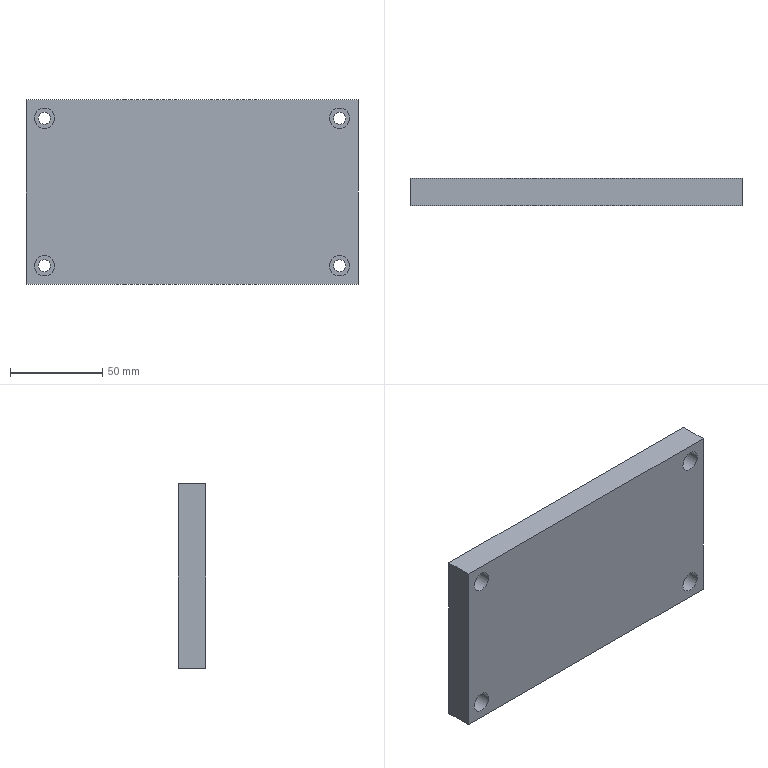Component | SolidWorks | SHYTJ-01-03-05-1 | 1 solid | 26 faces | box 180 x 15 x 100 mm | volume 266001 mm3 | cylinder 16 | plane 10 | commonest cylinder face diameters 11 x8 6.6 x8
build123d program:
from build123d import *

# Parameters (mm, degrees)
SKETCH1_W                                         = 180
SKETCH1_H                                         = 100
BOSS_EXTRUDE1_DEPTH                               = 15
HOLE_SIZE_ACCORDING_TO_TYPE_OF_SOCKET_D           = 6.6
HOLE_SIZE_ACCORDING_TO_TYPE_OF_SOCKET_DEPTH       = 19.75
HOLE_SIZE_ACCORDING_TO_TYPE_OF_SOCKET_CBORE_D     = 11
HOLE_SIZE_ACCORDING_TO_TYPE_OF_SOCKET_CBORE_DEPTH = 8
HOLE_SIZE_ACCORDING_TO_TYPE_OF_SOCKET_TIP         = 1.983


with BuildPart() as part:
    # Sketch1 → Boss-Extrude1 (new body)
    with BuildSketch(Plane.XY):
        with Locations((-90, -50)):
            Rectangle(SKETCH1_W, SKETCH1_H)
    extrude(amount=BOSS_EXTRUDE1_DEPTH)

    # Hole Size _according to_ type of socket
    with Locations(Plane(origin=(0, 0, 0), x_dir=(-1, 0, 0), z_dir=(0, 0, -1))):
        with Locations((10, -10), (10, -90), (170, -90), (170, -10)):
            CounterBoreHole(HOLE_SIZE_ACCORDING_TO_TYPE_OF_SOCKET_D / 2, HOLE_SIZE_ACCORDING_TO_TYPE_OF_SOCKET_CBORE_D / 2, HOLE_SIZE_ACCORDING_TO_TYPE_OF_SOCKET_CBORE_DEPTH, depth=HOLE_SIZE_ACCORDING_TO_TYPE_OF_SOCKET_DEPTH)
            with Locations((0, 0, -(HOLE_SIZE_ACCORDING_TO_TYPE_OF_SOCKET_DEPTH + HOLE_SIZE_ACCORDING_TO_TYPE_OF_SOCKET_TIP / 2))):  # 118° drill point
                Cone(0, HOLE_SIZE_ACCORDING_TO_TYPE_OF_SOCKET_D / 2, HOLE_SIZE_ACCORDING_TO_TYPE_OF_SOCKET_TIP, mode=Mode.SUBTRACT)


solid = part.part

# Placed as in the assembly
solid = solid.moved(Location((115.884, -80.361, 220), (-90, 0, 0)))
STEP:
#1=CARTESIAN_POINT('',(4.385,-2.849,9.055));
#2=VERTEX_POINT('',#1);
#3=CARTESIAN_POINT('',(3.952,-2.849,9.055));
#4=VERTEX_POINT('',#3);
#5=CARTESIAN_POINT('',(4.169,-2.849,9.055));
#6=DIRECTION('',(-0.,-1.,-0.));
#7=DIRECTION('',(-1.,0.,0.));
#8=AXIS2_PLACEMENT_3D('',#5,#6,#7);
#9=CIRCLE('',#8,0.2165);
#10=EDGE_CURVE('',#2,#4,#9,.T.);
#11=ORIENTED_EDGE('',*,*,#10,.F.);
#12=CARTESIAN_POINT('',(4.385,-3.164,9.055));
#13=VERTEX_POINT('',#12);
#14=CARTESIAN_POINT('',(4.385,-3.164,9.055));
#15=DIRECTION('',(-0.,-1.,-0.));
#16=VECTOR('',#15,39.37);
#17=LINE('',#14,#16);
#18=EDGE_CURVE('',#2,#13,#17,.T.);
#19=ORIENTED_EDGE('',*,*,#18,.T.);
#20=CARTESIAN_POINT('',(3.952,-3.164,9.055));
#21=VERTEX_POINT('',#20);
#22=CARTESIAN_POINT('',(4.169,-3.164,9.055));
#23=DIRECTION('',(-0.,-1.,-0.));
#24=DIRECTION('',(-1.,0.,0.));
#25=AXIS2_PLACEMENT_3D('',#22,#23,#24);
#26=CIRCLE('',#25,0.2165);
#27=EDGE_CURVE('',#13,#21,#26,.T.);
#28=ORIENTED_EDGE('',*,*,#27,.T.);
#29=CARTESIAN_POINT('',(3.952,-3.164,9.055));
#30=DIRECTION('',(-0.,-1.,-0.));
#31=VECTOR('',#30,39.37);
#32=LINE('',#29,#31);
#33=EDGE_CURVE('',#4,#21,#32,.T.);
#34=ORIENTED_EDGE('',*,*,#33,.F.);
#35=EDGE_LOOP('',(#11,#19,#28,#34));
#36=FACE_OUTER_BOUND('',#35,.T.);
#37=CARTESIAN_POINT('',(4.169,-3.164,9.055));
#38=DIRECTION('',(-0.,-1.,-0.));
#39=DIRECTION('',(-1.,0.,0.));
#40=AXIS2_PLACEMENT_3D('',#37,#38,#39);
#41=CYLINDRICAL_SURFACE('',#40,0.2165);
#42=ADVANCED_FACE('',(#36),#41,.F.);
#43=CARTESIAN_POINT('',(4.299,-2.573,9.055));
#44=VERTEX_POINT('',#43);
#45=CARTESIAN_POINT('',(4.039,-2.573,9.055));
#46=VERTEX_POINT('',#45);
#47=CARTESIAN_POINT('',(4.169,-2.573,9.055));
#48=DIRECTION('',(-0.,-1.,-0.));
#49=DIRECTION('',(-1.,0.,0.));
#50=AXIS2_PLACEMENT_3D('',#47,#48,#49);
#51=CIRCLE('',#50,0.1299);
#52=EDGE_CURVE('',#44,#46,#51,.T.);
#53=ORIENTED_EDGE('',*,*,#52,.F.);
#54=CARTESIAN_POINT('',(4.299,-2.849,9.055));
#55=VERTEX_POINT('',#54);
#56=CARTESIAN_POINT('',(4.299,-3.164,9.055));
#57=DIRECTION('',(-0.,-1.,-0.));
#58=VECTOR('',#57,39.37);
#59=LINE('',#56,#58);
#60=EDGE_CURVE('',#44,#55,#59,.T.);
#61=ORIENTED_EDGE('',*,*,#60,.T.);
#62=CARTESIAN_POINT('',(4.039,-2.849,9.055));
#63=VERTEX_POINT('',#62);
#64=CARTESIAN_POINT('',(4.169,-2.849,9.055));
#65=DIRECTION('',(-0.,-1.,-0.));
#66=DIRECTION('',(-1.,0.,0.));
#67=AXIS2_PLACEMENT_3D('',#64,#65,#66);
#68=CIRCLE('',#67,0.1299);
#69=EDGE_CURVE('',#55,#63,#68,.T.);
#70=ORIENTED_EDGE('',*,*,#69,.T.);
#71=CARTESIAN_POINT('',(4.039,-3.164,9.055));
#72=DIRECTION('',(-0.,-1.,-0.));
#73=VECTOR('',#72,39.37);
#74=LINE('',#71,#73);
#75=EDGE_CURVE('',#46,#63,#74,.T.);
#76=ORIENTED_EDGE('',*,*,#75,.F.);
#77=EDGE_LOOP('',(#53,#61,#70,#76));
#78=FACE_OUTER_BOUND('',#77,.T.);
#79=CARTESIAN_POINT('',(4.169,-3.164,9.055));
#80=DIRECTION('',(-0.,-1.,-0.));
#81=DIRECTION('',(-1.,0.,0.));
#82=AXIS2_PLACEMENT_3D('',#79,#80,#81);
#83=CYLINDRICAL_SURFACE('',#82,0.1299);
#84=ADVANCED_FACE('',(#78),#83,.F.);
#85=CARTESIAN_POINT('',(4.385,-2.849,12.205));
#86=VERTEX_POINT('',#85);
#87=CARTESIAN_POINT('',(3.952,-2.849,12.205));
#88=VERTEX_POINT('',#87);
#89=CARTESIAN_POINT('',(4.169,-2.849,12.205));
#90=DIRECTION('',(-0.,-1.,-0.));
#91=DIRECTION('',(-1.,0.,0.));
#92=AXIS2_PLACEMENT_3D('',#89,#90,#91);
#93=CIRCLE('',#92,0.2165);
#94=EDGE_CURVE('',#86,#88,#93,.T.);
#95=ORIENTED_EDGE('',*,*,#94,.F.);
#96=CARTESIAN_POINT('',(4.385,-3.164,12.205));
#97=VERTEX_POINT('',#96);
#98=CARTESIAN_POINT('',(4.385,-3.164,12.205));
#99=DIRECTION('',(-0.,-1.,-0.));
#100=VECTOR('',#99,39.37);
#101=LINE('',#98,#100);
#102=EDGE_CURVE('',#86,#97,#101,.T.);
#103=ORIENTED_EDGE('',*,*,#102,.T.);
#104=CARTESIAN_POINT('',(3.952,-3.164,12.205));
#105=VERTEX_POINT('',#104);
#106=CARTESIAN_POINT('',(4.169,-3.164,12.205));
#107=DIRECTION('',(-0.,-1.,-0.));
#108=DIRECTION('',(-1.,0.,0.));
#109=AXIS2_PLACEMENT_3D('',#106,#107,#108);
#110=CIRCLE('',#109,0.2165);
#111=EDGE_CURVE('',#97,#105,#110,.T.);
#112=ORIENTED_EDGE('',*,*,#111,.T.);
#113=CARTESIAN_POINT('',(3.952,-3.164,12.205));
#114=DIRECTION('',(-0.,-1.,-0.));
#115=VECTOR('',#114,39.37);
#116=LINE('',#113,#115);
#117=EDGE_CURVE('',#88,#105,#116,.T.);
#118=ORIENTED_EDGE('',*,*,#117,.F.);
#119=EDGE_LOOP('',(#95,#103,#112,#118));
#120=FACE_OUTER_BOUND('',#119,.T.);
#121=CARTESIAN_POINT('',(4.169,-3.164,12.205));
#122=DIRECTION('',(-0.,-1.,-0.));
#123=DIRECTION('',(-1.,0.,0.));
#124=AXIS2_PLACEMENT_3D('',#121,#122,#123);
#125=CYLINDRICAL_SURFACE('',#124,0.2165);
#126=ADVANCED_FACE('',(#120),#125,.F.);
#127=CARTESIAN_POINT('',(4.299,-2.573,12.205));
#128=VERTEX_POINT('',#127);
#129=CARTESIAN_POINT('',(4.039,-2.573,12.205));
#130=VERTEX_POINT('',#129);
#131=CARTESIAN_POINT('',(4.169,-2.573,12.205));
#132=DIRECTION('',(-0.,-1.,-0.));
#133=DIRECTION('',(-1.,0.,0.));
#134=AXIS2_PLACEMENT_3D('',#131,#132,#133);
#135=CIRCLE('',#134,0.1299);
#136=EDGE_CURVE('',#128,#130,#135,.T.);
#137=ORIENTED_EDGE('',*,*,#136,.F.);
#138=CARTESIAN_POINT('',(4.299,-2.849,12.205));
#139=VERTEX_POINT('',#138);
#140=CARTESIAN_POINT('',(4.299,-3.164,12.205));
#141=DIRECTION('',(-0.,-1.,-0.));
#142=VECTOR('',#141,39.37);
#143=LINE('',#140,#142);
#144=EDGE_CURVE('',#128,#139,#143,.T.);
#145=ORIENTED_EDGE('',*,*,#144,.T.);
#146=CARTESIAN_POINT('',(4.039,-2.849,12.205));
#147=VERTEX_POINT('',#146);
#148=CARTESIAN_POINT('',(4.169,-2.849,12.205));
#149=DIRECTION('',(-0.,-1.,-0.));
#150=DIRECTION('',(-1.,0.,0.));
#151=AXIS2_PLACEMENT_3D('',#148,#149,#150);
#152=CIRCLE('',#151,0.1299);
#153=EDGE_CURVE('',#139,#147,#152,.T.);
#154=ORIENTED_EDGE('',*,*,#153,.T.);
#155=CARTESIAN_POINT('',(4.039,-3.164,12.205));
#156=DIRECTION('',(-0.,-1.,-0.));
#157=VECTOR('',#156,39.37);
#158=LINE('',#155,#157);
#159=EDGE_CURVE('',#130,#147,#158,.T.);
#160=ORIENTED_EDGE('',*,*,#159,.F.);
#161=EDGE_LOOP('',(#137,#145,#154,#160));
#162=FACE_OUTER_BOUND('',#161,.T.);
#163=CARTESIAN_POINT('',(4.169,-3.164,12.205));
#164=DIRECTION('',(-0.,-1.,-0.));
#165=DIRECTION('',(-1.,0.,0.));
#166=AXIS2_PLACEMENT_3D('',#163,#164,#165);
#167=CYLINDRICAL_SURFACE('',#166,0.1299);
#168=ADVANCED_FACE('',(#162),#167,.F.);
#169=CARTESIAN_POINT('',(-1.914,-2.849,12.205));
#170=VERTEX_POINT('',#169);
#171=CARTESIAN_POINT('',(-2.347,-2.849,12.205));
#172=VERTEX_POINT('',#171);
#173=CARTESIAN_POINT('',(-2.131,-2.849,12.205));
#174=DIRECTION('',(-0.,-1.,-0.));
#175=DIRECTION('',(-1.,0.,0.));
#176=AXIS2_PLACEMENT_3D('',#173,#174,#175);
#177=CIRCLE('',#176,0.2165);
#178=EDGE_CURVE('',#170,#172,#177,.T.);
#179=ORIENTED_EDGE('',*,*,#178,.F.);
#180=CARTESIAN_POINT('',(-1.914,-3.164,12.205));
#181=VERTEX_POINT('',#180);
#182=CARTESIAN_POINT('',(-1.914,-3.164,12.205));
#183=DIRECTION('',(-0.,-1.,-0.));
#184=VECTOR('',#183,39.37);
#185=LINE('',#182,#184);
#186=EDGE_CURVE('',#170,#181,#185,.T.);
#187=ORIENTED_EDGE('',*,*,#186,.T.);
#188=CARTESIAN_POINT('',(-2.347,-3.164,12.205));
#189=VERTEX_POINT('',#188);
#190=CARTESIAN_POINT('',(-2.131,-3.164,12.205));
#191=DIRECTION('',(-0.,-1.,-0.));
#192=DIRECTION('',(-1.,0.,0.));
#193=AXIS2_PLACEMENT_3D('',#190,#191,#192);
#194=CIRCLE('',#193,0.2165);
#195=EDGE_CURVE('',#181,#189,#194,.T.);
#196=ORIENTED_EDGE('',*,*,#195,.T.);
#197=CARTESIAN_POINT('',(-2.347,-3.164,12.205));
#198=DIRECTION('',(-0.,-1.,-0.));
#199=VECTOR('',#198,39.37);
#200=LINE('',#197,#199);
#201=EDGE_CURVE('',#172,#189,#200,.T.);
#202=ORIENTED_EDGE('',*,*,#201,.F.);
#203=EDGE_LOOP('',(#179,#187,#196,#202));
#204=FACE_OUTER_BOUND('',#203,.T.);
#205=CARTESIAN_POINT('',(-2.131,-3.164,12.205));
#206=DIRECTION('',(-0.,-1.,-0.));
#207=DIRECTION('',(-1.,0.,0.));
#208=AXIS2_PLACEMENT_3D('',#205,#206,#207);
#209=CYLINDRICAL_SURFACE('',#208,0.2165);
#210=ADVANCED_FACE('',(#204),#209,.F.);
#211=CARTESIAN_POINT('',(-2.001,-2.573,12.205));
#212=VERTEX_POINT('',#211);
#213=CARTESIAN_POINT('',(-2.26,-2.573,12.205));
#214=VERTEX_POINT('',#213);
#215=CARTESIAN_POINT('',(-2.131,-2.573,12.205));
#216=DIRECTION('',(-0.,-1.,-0.));
#217=DIRECTION('',(-1.,0.,0.));
#218=AXIS2_PLACEMENT_3D('',#215,#216,#217);
#219=CIRCLE('',#218,0.1299);
#220=EDGE_CURVE('',#212,#214,#219,.T.);
#221=ORIENTED_EDGE('',*,*,#220,.F.);
#222=CARTESIAN_POINT('',(-2.001,-2.849,12.205));
#223=VERTEX_POINT('',#222);
#224=CARTESIAN_POINT('',(-2.001,-3.164,12.205));
#225=DIRECTION('',(-0.,-1.,-0.));
#226=VECTOR('',#225,39.37);
#227=LINE('',#224,#226);
#228=EDGE_CURVE('',#212,#223,#227,.T.);
#229=ORIENTED_EDGE('',*,*,#228,.T.);
#230=CARTESIAN_POINT('',(-2.26,-2.849,12.205));
#231=VERTEX_POINT('',#230);
#232=CARTESIAN_POINT('',(-2.131,-2.849,12.205));
#233=DIRECTION('',(-0.,-1.,-0.));
#234=DIRECTION('',(-1.,0.,0.));
#235=AXIS2_PLACEMENT_3D('',#232,#233,#234);
#236=CIRCLE('',#235,0.1299);
#237=EDGE_CURVE('',#223,#231,#236,.T.);
#238=ORIENTED_EDGE('',*,*,#237,.T.);
#239=CARTESIAN_POINT('',(-2.26,-3.164,12.205));
#240=DIRECTION('',(-0.,-1.,-0.));
#241=VECTOR('',#240,39.37);
#242=LINE('',#239,#241);
#243=EDGE_CURVE('',#214,#231,#242,.T.);
#244=ORIENTED_EDGE('',*,*,#243,.F.);
#245=EDGE_LOOP('',(#221,#229,#238,#244));
#246=FACE_OUTER_BOUND('',#245,.T.);
#247=CARTESIAN_POINT('',(-2.131,-3.164,12.205));
#248=DIRECTION('',(-0.,-1.,-0.));
#249=DIRECTION('',(-1.,0.,0.));
#250=AXIS2_PLACEMENT_3D('',#247,#248,#249);
#251=CYLINDRICAL_SURFACE('',#250,0.1299);
#252=ADVANCED_FACE('',(#246),#251,.F.);
#253=CARTESIAN_POINT('',(-1.914,-2.849,9.055));
#254=VERTEX_POINT('',#253);
#255=CARTESIAN_POINT('',(-2.347,-2.849,9.055));
#256=VERTEX_POINT('',#255);
#257=CARTESIAN_POINT('',(-2.131,-2.849,9.055));
#258=DIRECTION('',(-0.,-1.,-0.));
#259=DIRECTION('',(-1.,0.,0.));
#260=AXIS2_PLACEMENT_3D('',#257,#258,#259);
#261=CIRCLE('',#260,0.2165);
#262=EDGE_CURVE('',#254,#256,#261,.T.);
#263=ORIENTED_EDGE('',*,*,#262,.F.);
#264=CARTESIAN_POINT('',(-1.914,-3.164,9.055));
#265=VERTEX_POINT('',#264);
#266=CARTESIAN_POINT('',(-1.914,-3.164,9.055));
#267=DIRECTION('',(-0.,-1.,-0.));
#268=VECTOR('',#267,39.37);
#269=LINE('',#266,#268);
#270=EDGE_CURVE('',#254,#265,#269,.T.);
#271=ORIENTED_EDGE('',*,*,#270,.T.);
#272=CARTESIAN_POINT('',(-2.347,-3.164,9.055));
#273=VERTEX_POINT('',#272);
#274=CARTESIAN_POINT('',(-2.131,-3.164,9.055));
#275=DIRECTION('',(-0.,-1.,-0.));
#276=DIRECTION('',(-1.,0.,0.));
#277=AXIS2_PLACEMENT_3D('',#274,#275,#276);
#278=CIRCLE('',#277,0.2165);
#279=EDGE_CURVE('',#265,#273,#278,.T.);
#280=ORIENTED_EDGE('',*,*,#279,.T.);
#281=CARTESIAN_POINT('',(-2.347,-3.164,9.055));
#282=DIRECTION('',(-0.,-1.,-0.));
#283=VECTOR('',#282,39.37);
#284=LINE('',#281,#283);
#285=EDGE_CURVE('',#256,#273,#284,.T.);
#286=ORIENTED_EDGE('',*,*,#285,.F.);
#287=EDGE_LOOP('',(#263,#271,#280,#286));
#288=FACE_OUTER_BOUND('',#287,.T.);
#289=CARTESIAN_POINT('',(-2.131,-3.164,9.055));
#290=DIRECTION('',(-0.,-1.,-0.));
#291=DIRECTION('',(-1.,0.,0.));
#292=AXIS2_PLACEMENT_3D('',#289,#290,#291);
#293=CYLINDRICAL_SURFACE('',#292,0.2165);
#294=ADVANCED_FACE('',(#288),#293,.F.);
#295=CARTESIAN_POINT('',(-2.001,-2.573,9.055));
#296=VERTEX_POINT('',#295);
#297=CARTESIAN_POINT('',(-2.26,-2.573,9.055));
#298=VERTEX_POINT('',#297);
#299=CARTESIAN_POINT('',(-2.131,-2.573,9.055));
#300=DIRECTION('',(-0.,-1.,-0.));
#301=DIRECTION('',(-1.,0.,0.));
#302=AXIS2_PLACEMENT_3D('',#299,#300,#301);
#303=CIRCLE('',#302,0.1299);
#304=EDGE_CURVE('',#296,#298,#303,.T.);
#305=ORIENTED_EDGE('',*,*,#304,.F.);
#306=CARTESIAN_POINT('',(-2.001,-2.849,9.055));
#307=VERTEX_POINT('',#306);
#308=CARTESIAN_POINT('',(-2.001,-3.164,9.055));
#309=DIRECTION('',(-0.,-1.,-0.));
#310=VECTOR('',#309,39.37);
#311=LINE('',#308,#310);
#312=EDGE_CURVE('',#296,#307,#311,.T.);
#313=ORIENTED_EDGE('',*,*,#312,.T.);
#314=CARTESIAN_POINT('',(-2.26,-2.849,9.055));
#315=VERTEX_POINT('',#314);
#316=CARTESIAN_POINT('',(-2.131,-2.849,9.055));
#317=DIRECTION('',(-0.,-1.,-0.));
#318=DIRECTION('',(-1.,0.,0.));
#319=AXIS2_PLACEMENT_3D('',#316,#317,#318);
#320=CIRCLE('',#319,0.1299);
#321=EDGE_CURVE('',#307,#315,#320,.T.);
#322=ORIENTED_EDGE('',*,*,#321,.T.);
#323=CARTESIAN_POINT('',(-2.26,-3.164,9.055));
#324=DIRECTION('',(-0.,-1.,-0.));
#325=VECTOR('',#324,39.37);
#326=LINE('',#323,#325);
#327=EDGE_CURVE('',#298,#315,#326,.T.);
#328=ORIENTED_EDGE('',*,*,#327,.F.);
#329=EDGE_LOOP('',(#305,#313,#322,#328));
#330=FACE_OUTER_BOUND('',#329,.T.);
#331=CARTESIAN_POINT('',(-2.131,-3.164,9.055));
#332=DIRECTION('',(-0.,-1.,-0.));
#333=DIRECTION('',(-1.,0.,0.));
#334=AXIS2_PLACEMENT_3D('',#331,#332,#333);
#335=CYLINDRICAL_SURFACE('',#334,0.1299);
#336=ADVANCED_FACE('',(#330),#335,.F.);
#337=CARTESIAN_POINT('',(4.562,-3.164,12.598));
#338=VERTEX_POINT('',#337);
#339=CARTESIAN_POINT('',(4.562,-3.164,8.661));
#340=VERTEX_POINT('',#339);
#341=CARTESIAN_POINT('',(4.562,-3.164,8.661));
#342=DIRECTION('',(-0.,0.,-1.));
#343=VECTOR('',#342,39.37);
#344=LINE('',#341,#343);
#345=EDGE_CURVE('',#338,#340,#344,.T.);
#346=ORIENTED_EDGE('',*,*,#345,.T.);
#347=CARTESIAN_POINT('',(4.562,-2.573,8.661));
#348=VERTEX_POINT('',#347);
#349=CARTESIAN_POINT('',(4.562,-2.573,8.661));
#350=DIRECTION('',(-0.,-1.,-0.));
#351=VECTOR('',#350,39.37);
#352=LINE('',#349,#351);
#353=EDGE_CURVE('',#348,#340,#352,.T.);
#354=ORIENTED_EDGE('',*,*,#353,.F.);
#355=CARTESIAN_POINT('',(4.562,-2.573,12.598));
#356=VERTEX_POINT('',#355);
#357=CARTESIAN_POINT('',(4.562,-2.573,8.661));
#358=DIRECTION('',(-0.,0.,-1.));
#359=VECTOR('',#358,39.37);
#360=LINE('',#357,#359);
#361=EDGE_CURVE('',#356,#348,#360,.T.);
#362=ORIENTED_EDGE('',*,*,#361,.F.);
#363=CARTESIAN_POINT('',(4.562,-2.573,12.598));
#364=DIRECTION('',(-0.,-1.,-0.));
#365=VECTOR('',#364,39.37);
#366=LINE('',#363,#365);
#367=EDGE_CURVE('',#356,#338,#366,.T.);
#368=ORIENTED_EDGE('',*,*,#367,.T.);
#369=EDGE_LOOP('',(#346,#354,#362,#368));
#370=FACE_OUTER_BOUND('',#369,.T.);
#371=CARTESIAN_POINT('',(4.562,-2.573,8.661));
#372=DIRECTION('',(-1.,0.,0.));
#373=DIRECTION('',(0.,-0.,1.));
#374=AXIS2_PLACEMENT_3D('',#371,#372,#373);
#375=PLANE('',#374);
#376=ADVANCED_FACE('',(#370),#375,.F.);
#377=CARTESIAN_POINT('',(-2.524,-3.164,8.661));
#378=VERTEX_POINT('',#377);
#379=CARTESIAN_POINT('',(4.562,-3.164,8.661));
#380=DIRECTION('',(-1.,0.,0.));
#381=VECTOR('',#380,39.37);
#382=LINE('',#379,#381);
#383=EDGE_CURVE('',#340,#378,#382,.T.);
#384=ORIENTED_EDGE('',*,*,#383,.T.);
#385=CARTESIAN_POINT('',(-2.524,-2.573,8.661));
#386=VERTEX_POINT('',#385);
#387=CARTESIAN_POINT('',(-2.524,-2.573,8.661));
#388=DIRECTION('',(-0.,-1.,-0.));
#389=VECTOR('',#388,39.37);
#390=LINE('',#387,#389);
#391=EDGE_CURVE('',#386,#378,#390,.T.);
#392=ORIENTED_EDGE('',*,*,#391,.F.);
#393=CARTESIAN_POINT('',(4.562,-2.573,8.661));
#394=DIRECTION('',(-1.,0.,0.));
#395=VECTOR('',#394,39.37);
#396=LINE('',#393,#395);
#397=EDGE_CURVE('',#348,#386,#396,.T.);
#398=ORIENTED_EDGE('',*,*,#397,.F.);
#399=ORIENTED_EDGE('',*,*,#353,.T.);
#400=EDGE_LOOP('',(#384,#392,#398,#399));
#401=FACE_OUTER_BOUND('',#400,.T.);
#402=CARTESIAN_POINT('',(4.562,-2.573,8.661));
#403=DIRECTION('',(0.,-0.,1.));
#404=DIRECTION('',(1.,-0.,-0.));
#405=AXIS2_PLACEMENT_3D('',#402,#403,#404);
#406=PLANE('',#405);
#407=ADVANCED_FACE('',(#401),#406,.F.);
#408=CARTESIAN_POINT('',(-2.524,-3.164,12.598));
#409=VERTEX_POINT('',#408);
#410=CARTESIAN_POINT('',(-2.524,-3.164,8.661));
#411=DIRECTION('',(0.,-0.,1.));
#412=VECTOR('',#411,39.37);
#413=LINE('',#410,#412);
#414=EDGE_CURVE('',#378,#409,#413,.T.);
#415=ORIENTED_EDGE('',*,*,#414,.T.);
#416=CARTESIAN_POINT('',(-2.524,-2.573,12.598));
#417=VERTEX_POINT('',#416);
#418=CARTESIAN_POINT('',(-2.524,-2.573,12.598));
#419=DIRECTION('',(-0.,-1.,-0.));
#420=VECTOR('',#419,39.37);
#421=LINE('',#418,#420);
#422=EDGE_CURVE('',#417,#409,#421,.T.);
#423=ORIENTED_EDGE('',*,*,#422,.F.);
#424=CARTESIAN_POINT('',(-2.524,-2.573,8.661));
#425=DIRECTION('',(0.,-0.,1.));
#426=VECTOR('',#425,39.37);
#427=LINE('',#424,#426);
#428=EDGE_CURVE('',#386,#417,#427,.T.);
#429=ORIENTED_EDGE('',*,*,#428,.F.);
#430=ORIENTED_EDGE('',*,*,#391,.T.);
#431=EDGE_LOOP('',(#415,#423,#429,#430));
#432=FACE_OUTER_BOUND('',#431,.T.);
#433=CARTESIAN_POINT('',(-2.524,-2.573,8.661));
#434=DIRECTION('',(1.,-0.,-0.));
#435=DIRECTION('',(-0.,-1.,-0.));
#436=AXIS2_PLACEMENT_3D('',#433,#434,#435);
#437=PLANE('',#436);
#438=ADVANCED_FACE('',(#432),#437,.F.);
#439=CARTESIAN_POINT('',(4.562,-3.164,12.598));
#440=DIRECTION('',(1.,-0.,-0.));
#441=VECTOR('',#440,39.37);
#442=LINE('',#439,#441);
#443=EDGE_CURVE('',#409,#338,#442,.T.);
#444=ORIENTED_EDGE('',*,*,#443,.T.);
#445=ORIENTED_EDGE('',*,*,#367,.F.);
#446=CARTESIAN_POINT('',(4.562,-2.573,12.598));
#447=DIRECTION('',(1.,-0.,-0.));
#448=VECTOR('',#447,39.37);
#449=LINE('',#446,#448);
#450=EDGE_CURVE('',#417,#356,#449,.T.);
#451=ORIENTED_EDGE('',*,*,#450,.F.);
#452=ORIENTED_EDGE('',*,*,#422,.T.);
#453=EDGE_LOOP('',(#444,#445,#451,#452));
#454=FACE_OUTER_BOUND('',#453,.T.);
#455=CARTESIAN_POINT('',(4.562,-2.573,12.598));
#456=DIRECTION('',(-0.,0.,-1.));
#457=DIRECTION('',(-1.,0.,0.));
#458=AXIS2_PLACEMENT_3D('',#455,#456,#457);
#459=PLANE('',#458);
#460=ADVANCED_FACE('',(#454),#459,.F.);
#461=CARTESIAN_POINT('',(4.169,-2.573,9.055));
#462=DIRECTION('',(-0.,-1.,-0.));
#463=DIRECTION('',(-1.,0.,0.));
#464=AXIS2_PLACEMENT_3D('',#461,#462,#463);
#465=CIRCLE('',#464,0.1299);
#466=EDGE_CURVE('',#46,#44,#465,.T.);
#467=ORIENTED_EDGE('',*,*,#466,.T.);
#468=ORIENTED_EDGE('',*,*,#52,.T.);
#469=EDGE_LOOP('',(#467,#468));
#470=FACE_BOUND('',#469,.T.);
#471=CARTESIAN_POINT('',(4.169,-2.573,12.205));
#472=DIRECTION('',(-0.,-1.,-0.));
#473=DIRECTION('',(-1.,0.,0.));
#474=AXIS2_PLACEMENT_3D('',#471,#472,#473);
#475=CIRCLE('',#474,0.1299);
#476=EDGE_CURVE('',#130,#128,#475,.T.);
#477=ORIENTED_EDGE('',*,*,#476,.T.);
#478=ORIENTED_EDGE('',*,*,#136,.T.);
#479=EDGE_LOOP('',(#477,#478));
#480=FACE_BOUND('',#479,.T.);
#481=CARTESIAN_POINT('',(-2.131,-2.573,12.205));
#482=DIRECTION('',(-0.,-1.,-0.));
#483=DIRECTION('',(-1.,0.,0.));
#484=AXIS2_PLACEMENT_3D('',#481,#482,#483);
#485=CIRCLE('',#484,0.1299);
#486=EDGE_CURVE('',#214,#212,#485,.T.);
#487=ORIENTED_EDGE('',*,*,#486,.T.);
#488=ORIENTED_EDGE('',*,*,#220,.T.);
#489=EDGE_LOOP('',(#487,#488));
#490=FACE_BOUND('',#489,.T.);
#491=CARTESIAN_POINT('',(-2.131,-2.573,9.055));
#492=DIRECTION('',(-0.,-1.,-0.));
#493=DIRECTION('',(-1.,0.,0.));
#494=AXIS2_PLACEMENT_3D('',#491,#492,#493);
#495=CIRCLE('',#494,0.1299);
#496=EDGE_CURVE('',#298,#296,#495,.T.);
#497=ORIENTED_EDGE('',*,*,#496,.T.);
#498=ORIENTED_EDGE('',*,*,#304,.T.);
#499=EDGE_LOOP('',(#497,#498));
#500=FACE_BOUND('',#499,.T.);
#501=ORIENTED_EDGE('',*,*,#361,.T.);
#502=ORIENTED_EDGE('',*,*,#397,.T.);
#503=ORIENTED_EDGE('',*,*,#428,.T.);
#504=ORIENTED_EDGE('',*,*,#450,.T.);
#505=EDGE_LOOP('',(#501,#502,#503,#504));
#506=FACE_OUTER_BOUND('',#505,.T.);
#507=CARTESIAN_POINT('',(4.562,-2.573,8.661));
#508=DIRECTION('',(-0.,-1.,-0.));
#509=DIRECTION('',(-1.,0.,0.));
#510=AXIS2_PLACEMENT_3D('',#507,#508,#509);
#511=PLANE('',#510);
#512=ADVANCED_FACE('',(#470,#480,#490,#500,#506),#511,.F.);
#513=CARTESIAN_POINT('',(4.169,-3.164,9.055));
#514=DIRECTION('',(-0.,-1.,-0.));
#515=DIRECTION('',(-1.,0.,0.));
#516=AXIS2_PLACEMENT_3D('',#513,#514,#515);
#517=CIRCLE('',#516,0.2165);
#518=EDGE_CURVE('',#21,#13,#517,.T.);
#519=ORIENTED_EDGE('',*,*,#518,.F.);
#520=ORIENTED_EDGE('',*,*,#27,.F.);
#521=EDGE_LOOP('',(#519,#520));
#522=FACE_BOUND('',#521,.T.);
#523=CARTESIAN_POINT('',(4.169,-3.164,12.205));
#524=DIRECTION('',(-0.,-1.,-0.));
#525=DIRECTION('',(-1.,0.,0.));
#526=AXIS2_PLACEMENT_3D('',#523,#524,#525);
#527=CIRCLE('',#526,0.2165);
#528=EDGE_CURVE('',#105,#97,#527,.T.);
#529=ORIENTED_EDGE('',*,*,#528,.F.);
#530=ORIENTED_EDGE('',*,*,#111,.F.);
#531=EDGE_LOOP('',(#529,#530));
#532=FACE_BOUND('',#531,.T.);
#533=CARTESIAN_POINT('',(-2.131,-3.164,12.205));
#534=DIRECTION('',(-0.,-1.,-0.));
#535=DIRECTION('',(-1.,0.,0.));
#536=AXIS2_PLACEMENT_3D('',#533,#534,#535);
#537=CIRCLE('',#536,0.2165);
#538=EDGE_CURVE('',#189,#181,#537,.T.);
#539=ORIENTED_EDGE('',*,*,#538,.F.);
#540=ORIENTED_EDGE('',*,*,#195,.F.);
#541=EDGE_LOOP('',(#539,#540));
#542=FACE_BOUND('',#541,.T.);
#543=CARTESIAN_POINT('',(-2.131,-3.164,9.055));
#544=DIRECTION('',(-0.,-1.,-0.));
#545=DIRECTION('',(-1.,0.,0.));
#546=AXIS2_PLACEMENT_3D('',#543,#544,#545);
#547=CIRCLE('',#546,0.2165);
#548=EDGE_CURVE('',#273,#265,#547,.T.);
#549=ORIENTED_EDGE('',*,*,#548,.F.);
#550=ORIENTED_EDGE('',*,*,#279,.F.);
#551=EDGE_LOOP('',(#549,#550));
#552=FACE_BOUND('',#551,.T.);
#553=ORIENTED_EDGE('',*,*,#345,.F.);
#554=ORIENTED_EDGE('',*,*,#443,.F.);
#555=ORIENTED_EDGE('',*,*,#414,.F.);
#556=ORIENTED_EDGE('',*,*,#383,.F.);
#557=EDGE_LOOP('',(#553,#554,#555,#556));
#558=FACE_OUTER_BOUND('',#557,.T.);
#559=CARTESIAN_POINT('',(4.562,-3.164,8.661));
#560=DIRECTION('',(-0.,-1.,-0.));
#561=DIRECTION('',(-1.,0.,0.));
#562=AXIS2_PLACEMENT_3D('',#559,#560,#561);
#563=PLANE('',#562);
#564=ADVANCED_FACE('',(#522,#532,#542,#552,#558),#563,.T.);
#565=ORIENTED_EDGE('',*,*,#312,.F.);
#566=ORIENTED_EDGE('',*,*,#496,.F.);
#567=ORIENTED_EDGE('',*,*,#327,.T.);
#568=CARTESIAN_POINT('',(-2.131,-2.849,9.055));
#569=DIRECTION('',(-0.,-1.,-0.));
#570=DIRECTION('',(-1.,0.,0.));
#571=AXIS2_PLACEMENT_3D('',#568,#569,#570);
#572=CIRCLE('',#571,0.1299);
#573=EDGE_CURVE('',#315,#307,#572,.T.);
#574=ORIENTED_EDGE('',*,*,#573,.T.);
#575=EDGE_LOOP('',(#565,#566,#567,#574));
#576=FACE_OUTER_BOUND('',#575,.T.);
#577=CARTESIAN_POINT('',(-2.131,-3.164,9.055));
#578=DIRECTION('',(-0.,-1.,-0.));
#579=DIRECTION('',(-1.,0.,0.));
#580=AXIS2_PLACEMENT_3D('',#577,#578,#579);
#581=CYLINDRICAL_SURFACE('',#580,0.1299);
#582=ADVANCED_FACE('',(#576),#581,.F.);
#583=ORIENTED_EDGE('',*,*,#573,.F.);
#584=ORIENTED_EDGE('',*,*,#321,.F.);
#585=EDGE_LOOP('',(#583,#584));
#586=FACE_BOUND('',#585,.T.);
#587=CARTESIAN_POINT('',(-2.131,-2.849,9.055));
#588=DIRECTION('',(-0.,-1.,-0.));
#589=DIRECTION('',(-1.,0.,0.));
#590=AXIS2_PLACEMENT_3D('',#587,#588,#589);
#591=CIRCLE('',#590,0.2165);
#592=EDGE_CURVE('',#256,#254,#591,.T.);
#593=ORIENTED_EDGE('',*,*,#592,.T.);
#594=ORIENTED_EDGE('',*,*,#262,.T.);
#595=EDGE_LOOP('',(#593,#594));
#596=FACE_OUTER_BOUND('',#595,.T.);
#597=CARTESIAN_POINT('',(-2.001,-2.849,9.055));
#598=DIRECTION('',(0.,1.,0.));
#599=DIRECTION('',(1.,-0.,-0.));
#600=AXIS2_PLACEMENT_3D('',#597,#598,#599);
#601=PLANE('',#600);
#602=ADVANCED_FACE('',(#586,#596),#601,.F.);
#603=ORIENTED_EDGE('',*,*,#270,.F.);
#604=ORIENTED_EDGE('',*,*,#592,.F.);
#605=ORIENTED_EDGE('',*,*,#285,.T.);
#606=ORIENTED_EDGE('',*,*,#548,.T.);
#607=EDGE_LOOP('',(#603,#604,#605,#606));
#608=FACE_OUTER_BOUND('',#607,.T.);
#609=CARTESIAN_POINT('',(-2.131,-3.164,9.055));
#610=DIRECTION('',(-0.,-1.,-0.));
#611=DIRECTION('',(-1.,0.,0.));
#612=AXIS2_PLACEMENT_3D('',#609,#610,#611);
#613=CYLINDRICAL_SURFACE('',#612,0.2165);
#614=ADVANCED_FACE('',(#608),#613,.F.);
#615=ORIENTED_EDGE('',*,*,#228,.F.);
#616=ORIENTED_EDGE('',*,*,#486,.F.);
#617=ORIENTED_EDGE('',*,*,#243,.T.);
#618=CARTESIAN_POINT('',(-2.131,-2.849,12.205));
#619=DIRECTION('',(-0.,-1.,-0.));
#620=DIRECTION('',(-1.,0.,0.));
#621=AXIS2_PLACEMENT_3D('',#618,#619,#620);
#622=CIRCLE('',#621,0.1299);
#623=EDGE_CURVE('',#231,#223,#622,.T.);
#624=ORIENTED_EDGE('',*,*,#623,.T.);
#625=EDGE_LOOP('',(#615,#616,#617,#624));
#626=FACE_OUTER_BOUND('',#625,.T.);
#627=CARTESIAN_POINT('',(-2.131,-3.164,12.205));
#628=DIRECTION('',(-0.,-1.,-0.));
#629=DIRECTION('',(-1.,0.,0.));
#630=AXIS2_PLACEMENT_3D('',#627,#628,#629);
#631=CYLINDRICAL_SURFACE('',#630,0.1299);
#632=ADVANCED_FACE('',(#626),#631,.F.);
#633=ORIENTED_EDGE('',*,*,#623,.F.);
#634=ORIENTED_EDGE('',*,*,#237,.F.);
#635=EDGE_LOOP('',(#633,#634));
#636=FACE_BOUND('',#635,.T.);
#637=CARTESIAN_POINT('',(-2.131,-2.849,12.205));
#638=DIRECTION('',(-0.,-1.,-0.));
#639=DIRECTION('',(-1.,0.,0.));
#640=AXIS2_PLACEMENT_3D('',#637,#638,#639);
#641=CIRCLE('',#640,0.2165);
#642=EDGE_CURVE('',#172,#170,#641,.T.);
#643=ORIENTED_EDGE('',*,*,#642,.T.);
#644=ORIENTED_EDGE('',*,*,#178,.T.);
#645=EDGE_LOOP('',(#643,#644));
#646=FACE_OUTER_BOUND('',#645,.T.);
#647=CARTESIAN_POINT('',(-2.001,-2.849,12.205));
#648=DIRECTION('',(0.,1.,0.));
#649=DIRECTION('',(1.,-0.,-0.));
#650=AXIS2_PLACEMENT_3D('',#647,#648,#649);
#651=PLANE('',#650);
#652=ADVANCED_FACE('',(#636,#646),#651,.F.);
#653=ORIENTED_EDGE('',*,*,#186,.F.);
#654=ORIENTED_EDGE('',*,*,#642,.F.);
#655=ORIENTED_EDGE('',*,*,#201,.T.);
#656=ORIENTED_EDGE('',*,*,#538,.T.);
#657=EDGE_LOOP('',(#653,#654,#655,#656));
#658=FACE_OUTER_BOUND('',#657,.T.);
#659=CARTESIAN_POINT('',(-2.131,-3.164,12.205));
#660=DIRECTION('',(-0.,-1.,-0.));
#661=DIRECTION('',(-1.,0.,0.));
#662=AXIS2_PLACEMENT_3D('',#659,#660,#661);
#663=CYLINDRICAL_SURFACE('',#662,0.2165);
#664=ADVANCED_FACE('',(#658),#663,.F.);
#665=ORIENTED_EDGE('',*,*,#144,.F.);
#666=ORIENTED_EDGE('',*,*,#476,.F.);
#667=ORIENTED_EDGE('',*,*,#159,.T.);
#668=CARTESIAN_POINT('',(4.169,-2.849,12.205));
#669=DIRECTION('',(-0.,-1.,-0.));
#670=DIRECTION('',(-1.,0.,0.));
#671=AXIS2_PLACEMENT_3D('',#668,#669,#670);
#672=CIRCLE('',#671,0.1299);
#673=EDGE_CURVE('',#147,#139,#672,.T.);
#674=ORIENTED_EDGE('',*,*,#673,.T.);
#675=EDGE_LOOP('',(#665,#666,#667,#674));
#676=FACE_OUTER_BOUND('',#675,.T.);
#677=CARTESIAN_POINT('',(4.169,-3.164,12.205));
#678=DIRECTION('',(-0.,-1.,-0.));
#679=DIRECTION('',(-1.,0.,0.));
#680=AXIS2_PLACEMENT_3D('',#677,#678,#679);
#681=CYLINDRICAL_SURFACE('',#680,0.1299);
#682=ADVANCED_FACE('',(#676),#681,.F.);
#683=ORIENTED_EDGE('',*,*,#673,.F.);
#684=ORIENTED_EDGE('',*,*,#153,.F.);
#685=EDGE_LOOP('',(#683,#684));
#686=FACE_BOUND('',#685,.T.);
#687=CARTESIAN_POINT('',(4.169,-2.849,12.205));
#688=DIRECTION('',(-0.,-1.,-0.));
#689=DIRECTION('',(-1.,0.,0.));
#690=AXIS2_PLACEMENT_3D('',#687,#688,#689);
#691=CIRCLE('',#690,0.2165);
#692=EDGE_CURVE('',#88,#86,#691,.T.);
#693=ORIENTED_EDGE('',*,*,#692,.T.);
#694=ORIENTED_EDGE('',*,*,#94,.T.);
#695=EDGE_LOOP('',(#693,#694));
#696=FACE_OUTER_BOUND('',#695,.T.);
#697=CARTESIAN_POINT('',(4.299,-2.849,12.205));
#698=DIRECTION('',(0.,1.,0.));
#699=DIRECTION('',(1.,-0.,-0.));
#700=AXIS2_PLACEMENT_3D('',#697,#698,#699);
#701=PLANE('',#700);
#702=ADVANCED_FACE('',(#686,#696),#701,.F.);
#703=ORIENTED_EDGE('',*,*,#102,.F.);
#704=ORIENTED_EDGE('',*,*,#692,.F.);
#705=ORIENTED_EDGE('',*,*,#117,.T.);
#706=ORIENTED_EDGE('',*,*,#528,.T.);
#707=EDGE_LOOP('',(#703,#704,#705,#706));
#708=FACE_OUTER_BOUND('',#707,.T.);
#709=CARTESIAN_POINT('',(4.169,-3.164,12.205));
#710=DIRECTION('',(-0.,-1.,-0.));
#711=DIRECTION('',(-1.,0.,0.));
#712=AXIS2_PLACEMENT_3D('',#709,#710,#711);
#713=CYLINDRICAL_SURFACE('',#712,0.2165);
#714=ADVANCED_FACE('',(#708),#713,.F.);
#715=ORIENTED_EDGE('',*,*,#60,.F.);
#716=ORIENTED_EDGE('',*,*,#466,.F.);
#717=ORIENTED_EDGE('',*,*,#75,.T.);
#718=CARTESIAN_POINT('',(4.169,-2.849,9.055));
#719=DIRECTION('',(-0.,-1.,-0.));
#720=DIRECTION('',(-1.,0.,0.));
#721=AXIS2_PLACEMENT_3D('',#718,#719,#720);
#722=CIRCLE('',#721,0.1299);
#723=EDGE_CURVE('',#63,#55,#722,.T.);
#724=ORIENTED_EDGE('',*,*,#723,.T.);
#725=EDGE_LOOP('',(#715,#716,#717,#724));
#726=FACE_OUTER_BOUND('',#725,.T.);
#727=CARTESIAN_POINT('',(4.169,-3.164,9.055));
#728=DIRECTION('',(-0.,-1.,-0.));
#729=DIRECTION('',(-1.,0.,0.));
#730=AXIS2_PLACEMENT_3D('',#727,#728,#729);
#731=CYLINDRICAL_SURFACE('',#730,0.1299);
#732=ADVANCED_FACE('',(#726),#731,.F.);
#733=ORIENTED_EDGE('',*,*,#723,.F.);
#734=ORIENTED_EDGE('',*,*,#69,.F.);
#735=EDGE_LOOP('',(#733,#734));
#736=FACE_BOUND('',#735,.T.);
#737=CARTESIAN_POINT('',(4.169,-2.849,9.055));
#738=DIRECTION('',(-0.,-1.,-0.));
#739=DIRECTION('',(-1.,0.,0.));
#740=AXIS2_PLACEMENT_3D('',#737,#738,#739);
#741=CIRCLE('',#740,0.2165);
#742=EDGE_CURVE('',#4,#2,#741,.T.);
#743=ORIENTED_EDGE('',*,*,#742,.T.);
#744=ORIENTED_EDGE('',*,*,#10,.T.);
#745=EDGE_LOOP('',(#743,#744));
#746=FACE_OUTER_BOUND('',#745,.T.);
#747=CARTESIAN_POINT('',(4.299,-2.849,9.055));
#748=DIRECTION('',(0.,1.,0.));
#749=DIRECTION('',(1.,-0.,-0.));
#750=AXIS2_PLACEMENT_3D('',#747,#748,#749);
#751=PLANE('',#750);
#752=ADVANCED_FACE('',(#736,#746),#751,.F.);
#753=ORIENTED_EDGE('',*,*,#18,.F.);
#754=ORIENTED_EDGE('',*,*,#742,.F.);
#755=ORIENTED_EDGE('',*,*,#33,.T.);
#756=ORIENTED_EDGE('',*,*,#518,.T.);
#757=EDGE_LOOP('',(#753,#754,#755,#756));
#758=FACE_OUTER_BOUND('',#757,.T.);
#759=CARTESIAN_POINT('',(4.169,-3.164,9.055));
#760=DIRECTION('',(-0.,-1.,-0.));
#761=DIRECTION('',(-1.,0.,0.));
#762=AXIS2_PLACEMENT_3D('',#759,#760,#761);
#763=CYLINDRICAL_SURFACE('',#762,0.2165);
#764=ADVANCED_FACE('',(#758),#763,.F.);
#765=CLOSED_SHELL('',(#42,#84,#126,#168,#210,#252,#294,#336,#376,#407,#438,#460,#512,#564,#582,#602,#614,#632,#652,#664,#682,#702,#714,#732,#752,#764));
#766=MANIFOLD_SOLID_BREP('',#765);
#767=CARTESIAN_POINT('',(0.,0.,0.));
#768=DIRECTION('',(0.,0.,1.));
#769=DIRECTION('',(1.,0.,0.));
#770=AXIS2_PLACEMENT_3D('',#767,#768,#769);
#771=(LENGTH_UNIT()NAMED_UNIT(*)SI_UNIT($,.METRE.));
#772=LENGTH_MEASURE_WITH_UNIT(LENGTH_MEASURE(0.0254),#771);
#773=DIMENSIONAL_EXPONENTS(1.,0.,0.,0.,0.,0.,0.);
#774=(CONVERSION_BASED_UNIT('',#772)LENGTH_UNIT()NAMED_UNIT(#773));
#775=UNCERTAINTY_MEASURE_WITH_UNIT(LENGTH_MEASURE(0.00001),#774,'','');
#776=(NAMED_UNIT(*)PLANE_ANGLE_UNIT()SI_UNIT($,.RADIAN.));
#777=(NAMED_UNIT(*)SI_UNIT($,.STERADIAN.)SOLID_ANGLE_UNIT());
#778=(GEOMETRIC_REPRESENTATION_CONTEXT(3)GLOBAL_UNCERTAINTY_ASSIGNED_CONTEXT((#775))GLOBAL_UNIT_ASSIGNED_CONTEXT((#774,#776,#777))REPRESENTATION_CONTEXT('',''));
#779=ADVANCED_BREP_SHAPE_REPRESENTATION('',(#766,#770),#778);
#780=COLOUR_RGB('',0.7922,0.8196,0.9333);
#781=FILL_AREA_STYLE_COLOUR('',#780);
#782=FILL_AREA_STYLE('',(#781));
#783=SURFACE_STYLE_FILL_AREA(#782);
#784=SURFACE_SIDE_STYLE('',(#783));
#785=SURFACE_STYLE_USAGE(.BOTH.,#784);
#786=PRESENTATION_STYLE_ASSIGNMENT((#785));
#787=STYLED_ITEM('',(#786),#766);
#788=(LENGTH_UNIT()NAMED_UNIT(*)SI_UNIT($,.METRE.));
#789=LENGTH_MEASURE_WITH_UNIT(LENGTH_MEASURE(0.0254),#788);
#790=DIMENSIONAL_EXPONENTS(1.,0.,0.,0.,0.,0.,0.);
#791=(CONVERSION_BASED_UNIT('',#789)LENGTH_UNIT()NAMED_UNIT(#790));
#792=UNCERTAINTY_MEASURE_WITH_UNIT(LENGTH_MEASURE(0.00001),#791,'','');
#793=(NAMED_UNIT(*)PLANE_ANGLE_UNIT()SI_UNIT($,.RADIAN.));
#794=(NAMED_UNIT(*)SI_UNIT($,.STERADIAN.)SOLID_ANGLE_UNIT());
#795=(GEOMETRIC_REPRESENTATION_CONTEXT(3)GLOBAL_UNCERTAINTY_ASSIGNED_CONTEXT((#792))GLOBAL_UNIT_ASSIGNED_CONTEXT((#791,#793,#794))REPRESENTATION_CONTEXT('',''));
#796=MECHANICAL_DESIGN_GEOMETRIC_PRESENTATION_REPRESENTATION('',(#787),#795);
#797=PRESENTATION_LAYER_ASSIGNMENT('','',(#787));